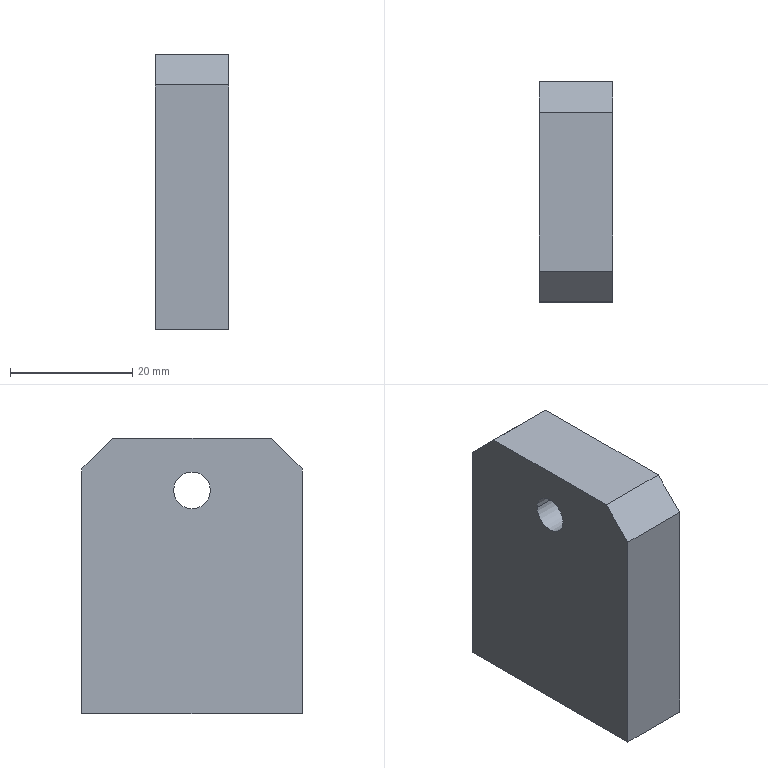Component | SolidWorks | 170423A4-ConveyorBeltIdlerAssembly1-1_170423A4-AdjustmentBlock2-1 | 1 solid | 18 faces | box 12 x 36 x 45 mm | volume 18598 mm3 | plane 8 | cylinder 6 | cone 4 | commonest cylinder face diameters 3.3 x4 6 x2
build123d program:
from build123d import *

# Parameters (mm, degrees)
SKETCH1_W             = 36
SKETCH1_H             = 45
BOSS_EXTRUDE1_DEPTH   = 12
CHAMFER1_SIZE         = 5
M6_TAPPED_HOLE1_D     = 6
M4_TAPPED_HOLE1_D     = 3.3
M4_TAPPED_HOLE1_DEPTH = 11.5
M4_TAPPED_HOLE1_TIP   = 0.9914


with BuildPart() as part:
    # Sketch1 → Boss-Extrude1 (new body)
    with BuildSketch(Plane.XY):
        with Locations((0, 22.5)):
            Rectangle(SKETCH1_W, SKETCH1_H)
    extrude(amount=BOSS_EXTRUDE1_DEPTH)

    # Chamfer1
    chamfer1_edges = [part.edges().sort_by_distance(p)[0] for p in [
        (-18, 45, 6),
        (18, 45, 6),
    ]]
    chamfer(chamfer1_edges, length=CHAMFER1_SIZE)

    # M6 Tapped Hole1 (through all)
    with Locations(Plane.XY.offset(12)):
        with Locations((0, 36.5)):
            Hole(M6_TAPPED_HOLE1_D / 2)

    # M4 Tapped Hole1
    with Locations(Plane(origin=(0, 0, 0), x_dir=(-1, 0, 0), z_dir=(0, -1, 0))):
        with Locations((12.5, -6), (-12.5, -6)):
            Hole(M4_TAPPED_HOLE1_D / 2, depth=M4_TAPPED_HOLE1_DEPTH)
            with Locations((0, 0, -(M4_TAPPED_HOLE1_DEPTH + M4_TAPPED_HOLE1_TIP / 2))):  # 118° drill point
                Cone(0, M4_TAPPED_HOLE1_D / 2, M4_TAPPED_HOLE1_TIP, mode=Mode.SUBTRACT)


solid = part.part

# Placed as in the assembly
solid = solid.moved(Location((-32.246, -95.788, 415), (90, -90, 0)))
STEP:
#1=CARTESIAN_POINT('',(-1.441,-3.279,16.791));
#2=VERTEX_POINT('',#1);
#3=CARTESIAN_POINT('',(-1.571,-3.279,16.791));
#4=VERTEX_POINT('',#3);
#5=CARTESIAN_POINT('',(-1.506,-3.279,16.791));
#6=DIRECTION('',(0.,-0.,-1.));
#7=DIRECTION('',(-1.,0.,0.));
#8=AXIS2_PLACEMENT_3D('',#5,#6,#7);
#9=CIRCLE('',#8,0.06496);
#10=EDGE_CURVE('',#2,#4,#9,.T.);
#11=ORIENTED_EDGE('',*,*,#10,.F.);
#12=CARTESIAN_POINT('',(-1.441,-3.279,16.339));
#13=VERTEX_POINT('',#12);
#14=CARTESIAN_POINT('',(-1.441,-3.279,16.339));
#15=DIRECTION('',(0.,-0.,-1.));
#16=VECTOR('',#15,39.37);
#17=LINE('',#14,#16);
#18=EDGE_CURVE('',#2,#13,#17,.T.);
#19=ORIENTED_EDGE('',*,*,#18,.T.);
#20=CARTESIAN_POINT('',(-1.571,-3.279,16.339));
#21=VERTEX_POINT('',#20);
#22=CARTESIAN_POINT('',(-1.506,-3.279,16.339));
#23=DIRECTION('',(0.,-0.,-1.));
#24=DIRECTION('',(-1.,0.,0.));
#25=AXIS2_PLACEMENT_3D('',#22,#23,#24);
#26=CIRCLE('',#25,0.06496);
#27=EDGE_CURVE('',#13,#21,#26,.T.);
#28=ORIENTED_EDGE('',*,*,#27,.T.);
#29=CARTESIAN_POINT('',(-1.571,-3.279,16.339));
#30=DIRECTION('',(0.,-0.,-1.));
#31=VECTOR('',#30,39.37);
#32=LINE('',#29,#31);
#33=EDGE_CURVE('',#4,#21,#32,.T.);
#34=ORIENTED_EDGE('',*,*,#33,.F.);
#35=EDGE_LOOP('',(#11,#19,#28,#34));
#36=FACE_OUTER_BOUND('',#35,.T.);
#37=CARTESIAN_POINT('',(-1.506,-3.279,16.339));
#38=DIRECTION('',(0.,-0.,-1.));
#39=DIRECTION('',(-1.,0.,0.));
#40=AXIS2_PLACEMENT_3D('',#37,#38,#39);
#41=CYLINDRICAL_SURFACE('',#40,0.06496);
#42=ADVANCED_FACE('',(#36),#41,.F.);
#43=CARTESIAN_POINT('',(-1.506,-3.279,16.83));
#44=VERTEX_POINT('',#43);
#45=CARTESIAN_POINT('',(-1.571,-3.279,16.791));
#46=DIRECTION('',(-0.8572,-0.,-0.515));
#47=VECTOR('',#46,39.37);
#48=LINE('',#45,#47);
#49=EDGE_CURVE('',#44,#4,#48,.T.);
#50=ORIENTED_EDGE('',*,*,#49,.F.);
#51=CARTESIAN_POINT('',(-1.441,-3.279,16.791));
#52=DIRECTION('',(0.8572,0.,-0.515));
#53=VECTOR('',#52,39.37);
#54=LINE('',#51,#53);
#55=EDGE_CURVE('',#44,#2,#54,.T.);
#56=ORIENTED_EDGE('',*,*,#55,.T.);
#57=ORIENTED_EDGE('',*,*,#10,.T.);
#58=EDGE_LOOP('',(#50,#56,#57));
#59=FACE_OUTER_BOUND('',#58,.T.);
#60=CARTESIAN_POINT('',(-1.506,-3.279,16.791));
#61=DIRECTION('',(0.,-0.,-1.));
#62=DIRECTION('',(-1.,0.,0.));
#63=AXIS2_PLACEMENT_3D('',#60,#61,#62);
#64=CONICAL_SURFACE('',#63,0.06496,1.03);
#65=ADVANCED_FACE('',(#59),#64,.F.);
#66=CARTESIAN_POINT('',(-1.441,-4.263,16.791));
#67=VERTEX_POINT('',#66);
#68=CARTESIAN_POINT('',(-1.571,-4.263,16.791));
#69=VERTEX_POINT('',#68);
#70=CARTESIAN_POINT('',(-1.506,-4.263,16.791));
#71=DIRECTION('',(0.,-0.,-1.));
#72=DIRECTION('',(-1.,0.,0.));
#73=AXIS2_PLACEMENT_3D('',#70,#71,#72);
#74=CIRCLE('',#73,0.06496);
#75=EDGE_CURVE('',#67,#69,#74,.T.);
#76=ORIENTED_EDGE('',*,*,#75,.F.);
#77=CARTESIAN_POINT('',(-1.441,-4.263,16.339));
#78=VERTEX_POINT('',#77);
#79=CARTESIAN_POINT('',(-1.441,-4.263,16.339));
#80=DIRECTION('',(0.,-0.,-1.));
#81=VECTOR('',#80,39.37);
#82=LINE('',#79,#81);
#83=EDGE_CURVE('',#67,#78,#82,.T.);
#84=ORIENTED_EDGE('',*,*,#83,.T.);
#85=CARTESIAN_POINT('',(-1.571,-4.263,16.339));
#86=VERTEX_POINT('',#85);
#87=CARTESIAN_POINT('',(-1.506,-4.263,16.339));
#88=DIRECTION('',(0.,-0.,-1.));
#89=DIRECTION('',(-1.,0.,0.));
#90=AXIS2_PLACEMENT_3D('',#87,#88,#89);
#91=CIRCLE('',#90,0.06496);
#92=EDGE_CURVE('',#78,#86,#91,.T.);
#93=ORIENTED_EDGE('',*,*,#92,.T.);
#94=CARTESIAN_POINT('',(-1.571,-4.263,16.339));
#95=DIRECTION('',(0.,-0.,-1.));
#96=VECTOR('',#95,39.37);
#97=LINE('',#94,#96);
#98=EDGE_CURVE('',#69,#86,#97,.T.);
#99=ORIENTED_EDGE('',*,*,#98,.F.);
#100=EDGE_LOOP('',(#76,#84,#93,#99));
#101=FACE_OUTER_BOUND('',#100,.T.);
#102=CARTESIAN_POINT('',(-1.506,-4.263,16.339));
#103=DIRECTION('',(0.,-0.,-1.));
#104=DIRECTION('',(-1.,0.,0.));
#105=AXIS2_PLACEMENT_3D('',#102,#103,#104);
#106=CYLINDRICAL_SURFACE('',#105,0.06496);
#107=ADVANCED_FACE('',(#101),#106,.F.);
#108=CARTESIAN_POINT('',(-1.506,-4.263,16.83));
#109=VERTEX_POINT('',#108);
#110=CARTESIAN_POINT('',(-1.571,-4.263,16.791));
#111=DIRECTION('',(-0.8572,-0.,-0.515));
#112=VECTOR('',#111,39.37);
#113=LINE('',#110,#112);
#114=EDGE_CURVE('',#109,#69,#113,.T.);
#115=ORIENTED_EDGE('',*,*,#114,.F.);
#116=CARTESIAN_POINT('',(-1.441,-4.263,16.791));
#117=DIRECTION('',(0.8572,0.,-0.515));
#118=VECTOR('',#117,39.37);
#119=LINE('',#116,#118);
#120=EDGE_CURVE('',#109,#67,#119,.T.);
#121=ORIENTED_EDGE('',*,*,#120,.T.);
#122=ORIENTED_EDGE('',*,*,#75,.T.);
#123=EDGE_LOOP('',(#115,#121,#122));
#124=FACE_OUTER_BOUND('',#123,.T.);
#125=CARTESIAN_POINT('',(-1.506,-4.263,16.791));
#126=DIRECTION('',(0.,-0.,-1.));
#127=DIRECTION('',(-1.,0.,0.));
#128=AXIS2_PLACEMENT_3D('',#125,#126,#127);
#129=CONICAL_SURFACE('',#128,0.06496,1.03);
#130=ADVANCED_FACE('',(#124),#129,.F.);
#131=CARTESIAN_POINT('',(-1.742,-3.889,17.776));
#132=VERTEX_POINT('',#131);
#133=CARTESIAN_POINT('',(-1.742,-3.653,17.776));
#134=VERTEX_POINT('',#133);
#135=CARTESIAN_POINT('',(-1.742,-3.771,17.776));
#136=DIRECTION('',(1.,0.,0.));
#137=DIRECTION('',(0.,1.,0.));
#138=AXIS2_PLACEMENT_3D('',#135,#136,#137);
#139=CIRCLE('',#138,0.1181);
#140=EDGE_CURVE('',#132,#134,#139,.T.);
#141=ORIENTED_EDGE('',*,*,#140,.F.);
#142=CARTESIAN_POINT('',(-1.27,-3.889,17.776));
#143=VERTEX_POINT('',#142);
#144=CARTESIAN_POINT('',(-1.27,-3.889,17.776));
#145=DIRECTION('',(1.,0.,0.));
#146=VECTOR('',#145,39.37);
#147=LINE('',#144,#146);
#148=EDGE_CURVE('',#132,#143,#147,.T.);
#149=ORIENTED_EDGE('',*,*,#148,.T.);
#150=CARTESIAN_POINT('',(-1.27,-3.653,17.776));
#151=VERTEX_POINT('',#150);
#152=CARTESIAN_POINT('',(-1.27,-3.771,17.776));
#153=DIRECTION('',(1.,0.,0.));
#154=DIRECTION('',(0.,1.,0.));
#155=AXIS2_PLACEMENT_3D('',#152,#153,#154);
#156=CIRCLE('',#155,0.1181);
#157=EDGE_CURVE('',#143,#151,#156,.T.);
#158=ORIENTED_EDGE('',*,*,#157,.T.);
#159=CARTESIAN_POINT('',(-1.27,-3.653,17.776));
#160=DIRECTION('',(1.,0.,0.));
#161=VECTOR('',#160,39.37);
#162=LINE('',#159,#161);
#163=EDGE_CURVE('',#134,#151,#162,.T.);
#164=ORIENTED_EDGE('',*,*,#163,.F.);
#165=EDGE_LOOP('',(#141,#149,#158,#164));
#166=FACE_OUTER_BOUND('',#165,.T.);
#167=CARTESIAN_POINT('',(-1.27,-3.771,17.776));
#168=DIRECTION('',(1.,0.,0.));
#169=DIRECTION('',(0.,1.,0.));
#170=AXIS2_PLACEMENT_3D('',#167,#168,#169);
#171=CYLINDRICAL_SURFACE('',#170,0.1181);
#172=ADVANCED_FACE('',(#166),#171,.F.);
#173=CARTESIAN_POINT('',(-1.27,-4.48,17.913));
#174=VERTEX_POINT('',#173);
#175=CARTESIAN_POINT('',(-1.27,-4.48,16.339));
#176=VERTEX_POINT('',#175);
#177=CARTESIAN_POINT('',(-1.27,-4.48,16.339));
#178=DIRECTION('',(0.,-0.,-1.));
#179=VECTOR('',#178,39.37);
#180=LINE('',#177,#179);
#181=EDGE_CURVE('',#174,#176,#180,.T.);
#182=ORIENTED_EDGE('',*,*,#181,.F.);
#183=CARTESIAN_POINT('',(-1.742,-4.48,17.913));
#184=VERTEX_POINT('',#183);
#185=CARTESIAN_POINT('',(-1.27,-4.48,17.913));
#186=DIRECTION('',(-1.,0.,0.));
#187=VECTOR('',#186,39.37);
#188=LINE('',#185,#187);
#189=EDGE_CURVE('',#174,#184,#188,.T.);
#190=ORIENTED_EDGE('',*,*,#189,.T.);
#191=CARTESIAN_POINT('',(-1.742,-4.48,16.339));
#192=VERTEX_POINT('',#191);
#193=CARTESIAN_POINT('',(-1.742,-4.48,16.339));
#194=DIRECTION('',(0.,-0.,-1.));
#195=VECTOR('',#194,39.37);
#196=LINE('',#193,#195);
#197=EDGE_CURVE('',#184,#192,#196,.T.);
#198=ORIENTED_EDGE('',*,*,#197,.T.);
#199=CARTESIAN_POINT('',(-1.27,-4.48,16.339));
#200=DIRECTION('',(-1.,0.,0.));
#201=VECTOR('',#200,39.37);
#202=LINE('',#199,#201);
#203=EDGE_CURVE('',#176,#192,#202,.T.);
#204=ORIENTED_EDGE('',*,*,#203,.F.);
#205=EDGE_LOOP('',(#182,#190,#198,#204));
#206=FACE_OUTER_BOUND('',#205,.T.);
#207=CARTESIAN_POINT('',(-1.27,-4.48,16.339));
#208=DIRECTION('',(0.,1.,-0.));
#209=DIRECTION('',(-1.,0.,0.));
#210=AXIS2_PLACEMENT_3D('',#207,#208,#209);
#211=PLANE('',#210);
#212=ADVANCED_FACE('',(#206),#211,.F.);
#213=CARTESIAN_POINT('',(-1.506,-3.279,16.339));
#214=DIRECTION('',(0.,-0.,-1.));
#215=DIRECTION('',(-1.,0.,0.));
#216=AXIS2_PLACEMENT_3D('',#213,#214,#215);
#217=CIRCLE('',#216,0.06496);
#218=EDGE_CURVE('',#21,#13,#217,.T.);
#219=ORIENTED_EDGE('',*,*,#218,.F.);
#220=ORIENTED_EDGE('',*,*,#27,.F.);
#221=EDGE_LOOP('',(#219,#220));
#222=FACE_BOUND('',#221,.T.);
#223=CARTESIAN_POINT('',(-1.506,-4.263,16.339));
#224=DIRECTION('',(0.,-0.,-1.));
#225=DIRECTION('',(-1.,0.,0.));
#226=AXIS2_PLACEMENT_3D('',#223,#224,#225);
#227=CIRCLE('',#226,0.06496);
#228=EDGE_CURVE('',#86,#78,#227,.T.);
#229=ORIENTED_EDGE('',*,*,#228,.F.);
#230=ORIENTED_EDGE('',*,*,#92,.F.);
#231=EDGE_LOOP('',(#229,#230));
#232=FACE_BOUND('',#231,.T.);
#233=CARTESIAN_POINT('',(-1.742,-3.063,16.339));
#234=VERTEX_POINT('',#233);
#235=CARTESIAN_POINT('',(-1.742,-4.48,16.339));
#236=DIRECTION('',(0.,1.,0.));
#237=VECTOR('',#236,39.37);
#238=LINE('',#235,#237);
#239=EDGE_CURVE('',#192,#234,#238,.T.);
#240=ORIENTED_EDGE('',*,*,#239,.T.);
#241=CARTESIAN_POINT('',(-1.27,-3.063,16.339));
#242=VERTEX_POINT('',#241);
#243=CARTESIAN_POINT('',(-1.27,-3.063,16.339));
#244=DIRECTION('',(-1.,0.,0.));
#245=VECTOR('',#244,39.37);
#246=LINE('',#243,#245);
#247=EDGE_CURVE('',#242,#234,#246,.T.);
#248=ORIENTED_EDGE('',*,*,#247,.F.);
#249=CARTESIAN_POINT('',(-1.27,-4.48,16.339));
#250=DIRECTION('',(0.,1.,0.));
#251=VECTOR('',#250,39.37);
#252=LINE('',#249,#251);
#253=EDGE_CURVE('',#176,#242,#252,.T.);
#254=ORIENTED_EDGE('',*,*,#253,.F.);
#255=ORIENTED_EDGE('',*,*,#203,.T.);
#256=EDGE_LOOP('',(#240,#248,#254,#255));
#257=FACE_OUTER_BOUND('',#256,.T.);
#258=CARTESIAN_POINT('',(-1.27,-4.48,16.339));
#259=DIRECTION('',(0.,-0.,1.));
#260=DIRECTION('',(0.,-1.,-0.));
#261=AXIS2_PLACEMENT_3D('',#258,#259,#260);
#262=PLANE('',#261);
#263=ADVANCED_FACE('',(#222,#232,#257),#262,.F.);
#264=CARTESIAN_POINT('',(-1.742,-3.063,17.913));
#265=VERTEX_POINT('',#264);
#266=CARTESIAN_POINT('',(-1.742,-3.063,16.339));
#267=DIRECTION('',(0.,-0.,1.));
#268=VECTOR('',#267,39.37);
#269=LINE('',#266,#268);
#270=EDGE_CURVE('',#234,#265,#269,.T.);
#271=ORIENTED_EDGE('',*,*,#270,.T.);
#272=CARTESIAN_POINT('',(-1.27,-3.063,17.913));
#273=VERTEX_POINT('',#272);
#274=CARTESIAN_POINT('',(-1.27,-3.063,17.913));
#275=DIRECTION('',(1.,0.,0.));
#276=VECTOR('',#275,39.37);
#277=LINE('',#274,#276);
#278=EDGE_CURVE('',#265,#273,#277,.T.);
#279=ORIENTED_EDGE('',*,*,#278,.T.);
#280=CARTESIAN_POINT('',(-1.27,-3.063,16.339));
#281=DIRECTION('',(0.,-0.,1.));
#282=VECTOR('',#281,39.37);
#283=LINE('',#280,#282);
#284=EDGE_CURVE('',#242,#273,#283,.T.);
#285=ORIENTED_EDGE('',*,*,#284,.F.);
#286=ORIENTED_EDGE('',*,*,#247,.T.);
#287=EDGE_LOOP('',(#271,#279,#285,#286));
#288=FACE_OUTER_BOUND('',#287,.T.);
#289=CARTESIAN_POINT('',(-1.27,-3.063,16.339));
#290=DIRECTION('',(0.,-1.,-0.));
#291=DIRECTION('',(0.,0.,-1.));
#292=AXIS2_PLACEMENT_3D('',#289,#290,#291);
#293=PLANE('',#292);
#294=ADVANCED_FACE('',(#288),#293,.F.);
#295=CARTESIAN_POINT('',(-1.27,-3.259,18.11));
#296=VERTEX_POINT('',#295);
#297=CARTESIAN_POINT('',(-1.27,-4.283,18.11));
#298=VERTEX_POINT('',#297);
#299=CARTESIAN_POINT('',(-1.27,-4.48,18.11));
#300=DIRECTION('',(0.,-1.,-0.));
#301=VECTOR('',#300,39.37);
#302=LINE('',#299,#301);
#303=EDGE_CURVE('',#296,#298,#302,.T.);
#304=ORIENTED_EDGE('',*,*,#303,.F.);
#305=CARTESIAN_POINT('',(-1.742,-3.259,18.11));
#306=VERTEX_POINT('',#305);
#307=CARTESIAN_POINT('',(-1.27,-3.259,18.11));
#308=DIRECTION('',(-1.,0.,0.));
#309=VECTOR('',#308,39.37);
#310=LINE('',#307,#309);
#311=EDGE_CURVE('',#296,#306,#310,.T.);
#312=ORIENTED_EDGE('',*,*,#311,.T.);
#313=CARTESIAN_POINT('',(-1.742,-4.283,18.11));
#314=VERTEX_POINT('',#313);
#315=CARTESIAN_POINT('',(-1.742,-4.48,18.11));
#316=DIRECTION('',(0.,-1.,-0.));
#317=VECTOR('',#316,39.37);
#318=LINE('',#315,#317);
#319=EDGE_CURVE('',#306,#314,#318,.T.);
#320=ORIENTED_EDGE('',*,*,#319,.T.);
#321=CARTESIAN_POINT('',(-1.27,-4.283,18.11));
#322=DIRECTION('',(1.,0.,0.));
#323=VECTOR('',#322,39.37);
#324=LINE('',#321,#323);
#325=EDGE_CURVE('',#314,#298,#324,.T.);
#326=ORIENTED_EDGE('',*,*,#325,.T.);
#327=EDGE_LOOP('',(#304,#312,#320,#326));
#328=FACE_OUTER_BOUND('',#327,.T.);
#329=CARTESIAN_POINT('',(-1.27,-4.48,18.11));
#330=DIRECTION('',(0.,0.,-1.));
#331=DIRECTION('',(0.,1.,0.));
#332=AXIS2_PLACEMENT_3D('',#329,#330,#331);
#333=PLANE('',#332);
#334=ADVANCED_FACE('',(#328),#333,.F.);
#335=CARTESIAN_POINT('',(-1.27,-3.771,17.776));
#336=DIRECTION('',(1.,0.,0.));
#337=DIRECTION('',(0.,1.,0.));
#338=AXIS2_PLACEMENT_3D('',#335,#336,#337);
#339=CIRCLE('',#338,0.1181);
#340=EDGE_CURVE('',#151,#143,#339,.T.);
#341=ORIENTED_EDGE('',*,*,#340,.F.);
#342=ORIENTED_EDGE('',*,*,#157,.F.);
#343=EDGE_LOOP('',(#341,#342));
#344=FACE_BOUND('',#343,.T.);
#345=ORIENTED_EDGE('',*,*,#284,.T.);
#346=CARTESIAN_POINT('',(-1.27,-3.259,18.11));
#347=DIRECTION('',(0.,-0.7071,0.7071));
#348=VECTOR('',#347,39.37);
#349=LINE('',#346,#348);
#350=EDGE_CURVE('',#273,#296,#349,.T.);
#351=ORIENTED_EDGE('',*,*,#350,.T.);
#352=ORIENTED_EDGE('',*,*,#303,.T.);
#353=CARTESIAN_POINT('',(-1.27,-4.48,17.913));
#354=DIRECTION('',(0.,-0.7071,-0.7071));
#355=VECTOR('',#354,39.37);
#356=LINE('',#353,#355);
#357=EDGE_CURVE('',#298,#174,#356,.T.);
#358=ORIENTED_EDGE('',*,*,#357,.T.);
#359=ORIENTED_EDGE('',*,*,#181,.T.);
#360=ORIENTED_EDGE('',*,*,#253,.T.);
#361=EDGE_LOOP('',(#345,#351,#352,#358,#359,#360));
#362=FACE_OUTER_BOUND('',#361,.T.);
#363=CARTESIAN_POINT('',(-1.27,-3.771,16.339));
#364=DIRECTION('',(-1.,0.,0.));
#365=DIRECTION('',(0.,-1.,0.));
#366=AXIS2_PLACEMENT_3D('',#363,#364,#365);
#367=PLANE('',#366);
#368=ADVANCED_FACE('',(#344,#362),#367,.F.);
#369=CARTESIAN_POINT('',(-1.742,-3.771,17.776));
#370=DIRECTION('',(1.,0.,0.));
#371=DIRECTION('',(0.,1.,0.));
#372=AXIS2_PLACEMENT_3D('',#369,#370,#371);
#373=CIRCLE('',#372,0.1181);
#374=EDGE_CURVE('',#134,#132,#373,.T.);
#375=ORIENTED_EDGE('',*,*,#374,.T.);
#376=ORIENTED_EDGE('',*,*,#140,.T.);
#377=EDGE_LOOP('',(#375,#376));
#378=FACE_BOUND('',#377,.T.);
#379=ORIENTED_EDGE('',*,*,#319,.F.);
#380=CARTESIAN_POINT('',(-1.742,-2.629,17.48));
#381=DIRECTION('',(0.,0.7071,-0.7071));
#382=VECTOR('',#381,39.37);
#383=LINE('',#380,#382);
#384=EDGE_CURVE('',#306,#265,#383,.T.);
#385=ORIENTED_EDGE('',*,*,#384,.T.);
#386=ORIENTED_EDGE('',*,*,#270,.F.);
#387=ORIENTED_EDGE('',*,*,#239,.F.);
#388=ORIENTED_EDGE('',*,*,#197,.F.);
#389=CARTESIAN_POINT('',(-1.742,-4.913,17.48));
#390=DIRECTION('',(0.,0.7071,0.7071));
#391=VECTOR('',#390,39.37);
#392=LINE('',#389,#391);
#393=EDGE_CURVE('',#184,#314,#392,.T.);
#394=ORIENTED_EDGE('',*,*,#393,.T.);
#395=EDGE_LOOP('',(#379,#385,#386,#387,#388,#394));
#396=FACE_OUTER_BOUND('',#395,.T.);
#397=CARTESIAN_POINT('',(-1.742,-3.771,16.339));
#398=DIRECTION('',(-1.,0.,0.));
#399=DIRECTION('',(0.,-1.,0.));
#400=AXIS2_PLACEMENT_3D('',#397,#398,#399);
#401=PLANE('',#400);
#402=ADVANCED_FACE('',(#378,#396),#401,.T.);
#403=ORIENTED_EDGE('',*,*,#350,.F.);
#404=ORIENTED_EDGE('',*,*,#278,.F.);
#405=ORIENTED_EDGE('',*,*,#384,.F.);
#406=ORIENTED_EDGE('',*,*,#311,.F.);
#407=EDGE_LOOP('',(#403,#404,#405,#406));
#408=FACE_OUTER_BOUND('',#407,.T.);
#409=CARTESIAN_POINT('',(-1.27,-3.259,18.11));
#410=DIRECTION('',(0.,-0.7071,-0.7071));
#411=DIRECTION('',(-1.,0.,0.));
#412=AXIS2_PLACEMENT_3D('',#409,#410,#411);
#413=PLANE('',#412);
#414=ADVANCED_FACE('',(#408),#413,.F.);
#415=ORIENTED_EDGE('',*,*,#357,.F.);
#416=ORIENTED_EDGE('',*,*,#325,.F.);
#417=ORIENTED_EDGE('',*,*,#393,.F.);
#418=ORIENTED_EDGE('',*,*,#189,.F.);
#419=EDGE_LOOP('',(#415,#416,#417,#418));
#420=FACE_OUTER_BOUND('',#419,.T.);
#421=CARTESIAN_POINT('',(-1.27,-4.48,17.913));
#422=DIRECTION('',(0.,0.7071,-0.7071));
#423=DIRECTION('',(-1.,0.,0.));
#424=AXIS2_PLACEMENT_3D('',#421,#422,#423);
#425=PLANE('',#424);
#426=ADVANCED_FACE('',(#420),#425,.F.);
#427=ORIENTED_EDGE('',*,*,#148,.F.);
#428=ORIENTED_EDGE('',*,*,#374,.F.);
#429=ORIENTED_EDGE('',*,*,#163,.T.);
#430=ORIENTED_EDGE('',*,*,#340,.T.);
#431=EDGE_LOOP('',(#427,#428,#429,#430));
#432=FACE_OUTER_BOUND('',#431,.T.);
#433=CARTESIAN_POINT('',(-1.27,-3.771,17.776));
#434=DIRECTION('',(1.,0.,0.));
#435=DIRECTION('',(0.,1.,0.));
#436=AXIS2_PLACEMENT_3D('',#433,#434,#435);
#437=CYLINDRICAL_SURFACE('',#436,0.1181);
#438=ADVANCED_FACE('',(#432),#437,.F.);
#439=ORIENTED_EDGE('',*,*,#120,.F.);
#440=ORIENTED_EDGE('',*,*,#114,.T.);
#441=CARTESIAN_POINT('',(-1.506,-4.263,16.791));
#442=DIRECTION('',(0.,-0.,-1.));
#443=DIRECTION('',(-1.,0.,0.));
#444=AXIS2_PLACEMENT_3D('',#441,#442,#443);
#445=CIRCLE('',#444,0.06496);
#446=EDGE_CURVE('',#69,#67,#445,.T.);
#447=ORIENTED_EDGE('',*,*,#446,.T.);
#448=EDGE_LOOP('',(#439,#440,#447));
#449=FACE_OUTER_BOUND('',#448,.T.);
#450=CARTESIAN_POINT('',(-1.506,-4.263,16.791));
#451=DIRECTION('',(0.,-0.,-1.));
#452=DIRECTION('',(-1.,0.,0.));
#453=AXIS2_PLACEMENT_3D('',#450,#451,#452);
#454=CONICAL_SURFACE('',#453,0.06496,1.03);
#455=ADVANCED_FACE('',(#449),#454,.F.);
#456=ORIENTED_EDGE('',*,*,#83,.F.);
#457=ORIENTED_EDGE('',*,*,#446,.F.);
#458=ORIENTED_EDGE('',*,*,#98,.T.);
#459=ORIENTED_EDGE('',*,*,#228,.T.);
#460=EDGE_LOOP('',(#456,#457,#458,#459));
#461=FACE_OUTER_BOUND('',#460,.T.);
#462=CARTESIAN_POINT('',(-1.506,-4.263,16.339));
#463=DIRECTION('',(0.,-0.,-1.));
#464=DIRECTION('',(-1.,0.,0.));
#465=AXIS2_PLACEMENT_3D('',#462,#463,#464);
#466=CYLINDRICAL_SURFACE('',#465,0.06496);
#467=ADVANCED_FACE('',(#461),#466,.F.);
#468=ORIENTED_EDGE('',*,*,#55,.F.);
#469=ORIENTED_EDGE('',*,*,#49,.T.);
#470=CARTESIAN_POINT('',(-1.506,-3.279,16.791));
#471=DIRECTION('',(0.,-0.,-1.));
#472=DIRECTION('',(-1.,0.,0.));
#473=AXIS2_PLACEMENT_3D('',#470,#471,#472);
#474=CIRCLE('',#473,0.06496);
#475=EDGE_CURVE('',#4,#2,#474,.T.);
#476=ORIENTED_EDGE('',*,*,#475,.T.);
#477=EDGE_LOOP('',(#468,#469,#476));
#478=FACE_OUTER_BOUND('',#477,.T.);
#479=CARTESIAN_POINT('',(-1.506,-3.279,16.791));
#480=DIRECTION('',(0.,-0.,-1.));
#481=DIRECTION('',(-1.,0.,0.));
#482=AXIS2_PLACEMENT_3D('',#479,#480,#481);
#483=CONICAL_SURFACE('',#482,0.06496,1.03);
#484=ADVANCED_FACE('',(#478),#483,.F.);
#485=ORIENTED_EDGE('',*,*,#18,.F.);
#486=ORIENTED_EDGE('',*,*,#475,.F.);
#487=ORIENTED_EDGE('',*,*,#33,.T.);
#488=ORIENTED_EDGE('',*,*,#218,.T.);
#489=EDGE_LOOP('',(#485,#486,#487,#488));
#490=FACE_OUTER_BOUND('',#489,.T.);
#491=CARTESIAN_POINT('',(-1.506,-3.279,16.339));
#492=DIRECTION('',(0.,-0.,-1.));
#493=DIRECTION('',(-1.,0.,0.));
#494=AXIS2_PLACEMENT_3D('',#491,#492,#493);
#495=CYLINDRICAL_SURFACE('',#494,0.06496);
#496=ADVANCED_FACE('',(#490),#495,.F.);
#497=CLOSED_SHELL('',(#42,#65,#107,#130,#172,#212,#263,#294,#334,#368,#402,#414,#426,#438,#455,#467,#484,#496));
#498=MANIFOLD_SOLID_BREP('',#497);
#499=CARTESIAN_POINT('',(0.,0.,0.));
#500=DIRECTION('',(0.,0.,1.));
#501=DIRECTION('',(1.,0.,0.));
#502=AXIS2_PLACEMENT_3D('',#499,#500,#501);
#503=(LENGTH_UNIT()NAMED_UNIT(*)SI_UNIT($,.METRE.));
#504=LENGTH_MEASURE_WITH_UNIT(LENGTH_MEASURE(0.0254),#503);
#505=DIMENSIONAL_EXPONENTS(1.,0.,0.,0.,0.,0.,0.);
#506=(CONVERSION_BASED_UNIT('',#504)LENGTH_UNIT()NAMED_UNIT(#505));
#507=UNCERTAINTY_MEASURE_WITH_UNIT(LENGTH_MEASURE(0.00001),#506,'','');
#508=(NAMED_UNIT(*)PLANE_ANGLE_UNIT()SI_UNIT($,.RADIAN.));
#509=(NAMED_UNIT(*)SI_UNIT($,.STERADIAN.)SOLID_ANGLE_UNIT());
#510=(GEOMETRIC_REPRESENTATION_CONTEXT(3)GLOBAL_UNCERTAINTY_ASSIGNED_CONTEXT((#507))GLOBAL_UNIT_ASSIGNED_CONTEXT((#506,#508,#509))REPRESENTATION_CONTEXT('',''));
#511=ADVANCED_BREP_SHAPE_REPRESENTATION('',(#498,#502),#510);
#512=COLOUR_RGB('',0.7922,0.8196,0.9333);
#513=FILL_AREA_STYLE_COLOUR('',#512);
#514=FILL_AREA_STYLE('',(#513));
#515=SURFACE_STYLE_FILL_AREA(#514);
#516=SURFACE_SIDE_STYLE('',(#515));
#517=SURFACE_STYLE_USAGE(.BOTH.,#516);
#518=PRESENTATION_STYLE_ASSIGNMENT((#517));
#519=STYLED_ITEM('',(#518),#498);
#520=(LENGTH_UNIT()NAMED_UNIT(*)SI_UNIT($,.METRE.));
#521=LENGTH_MEASURE_WITH_UNIT(LENGTH_MEASURE(0.0254),#520);
#522=DIMENSIONAL_EXPONENTS(1.,0.,0.,0.,0.,0.,0.);
#523=(CONVERSION_BASED_UNIT('',#521)LENGTH_UNIT()NAMED_UNIT(#522));
#524=UNCERTAINTY_MEASURE_WITH_UNIT(LENGTH_MEASURE(0.00001),#523,'','');
#525=(NAMED_UNIT(*)PLANE_ANGLE_UNIT()SI_UNIT($,.RADIAN.));
#526=(NAMED_UNIT(*)SI_UNIT($,.STERADIAN.)SOLID_ANGLE_UNIT());
#527=(GEOMETRIC_REPRESENTATION_CONTEXT(3)GLOBAL_UNCERTAINTY_ASSIGNED_CONTEXT((#524))GLOBAL_UNIT_ASSIGNED_CONTEXT((#523,#525,#526))REPRESENTATION_CONTEXT('',''));
#528=MECHANICAL_DESIGN_GEOMETRIC_PRESENTATION_REPRESENTATION('',(#519),#527);
#529=PRESENTATION_LAYER_ASSIGNMENT('','',(#519));